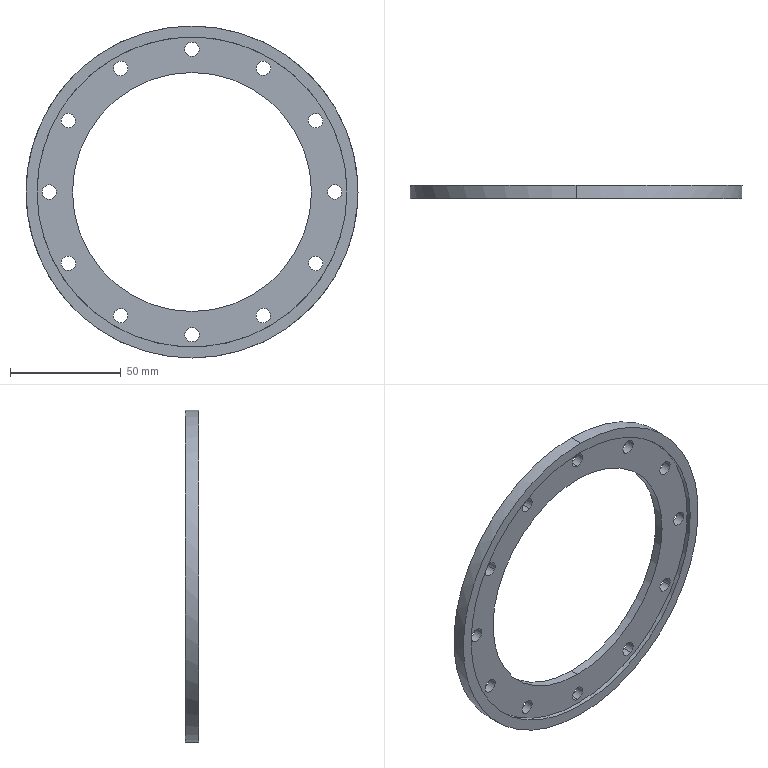CAM job | Mastercam | mm | 1 operations | part box 150 x 6 x 150
1. Drill/Counterbore | 7 - 4 倒角刀